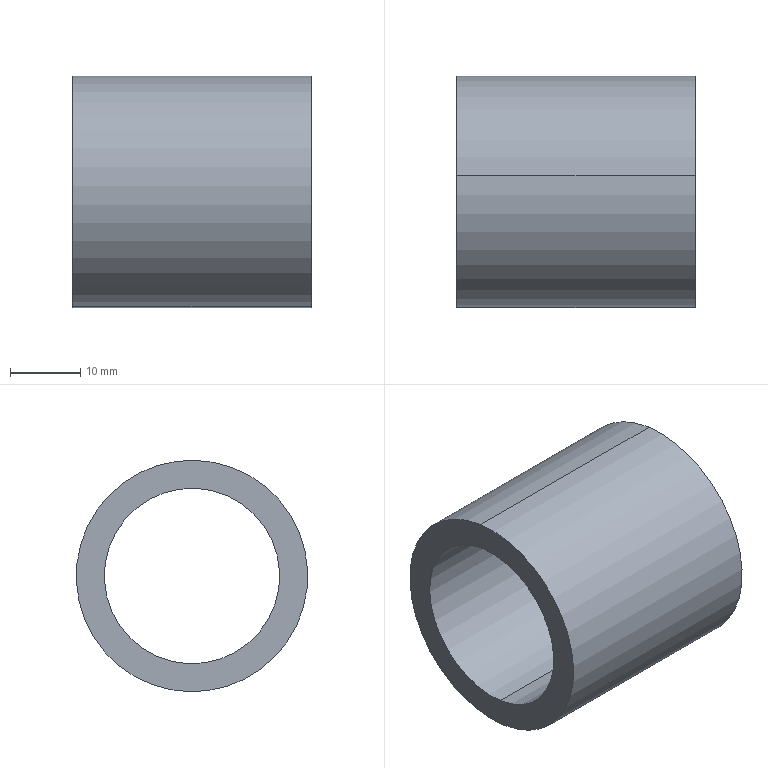Component | SolidWorks | 4-12-12ClampingAxisAssembly-1_4-12-7ClampingAxisBearingInnerPad-1 | 1 solid | 6 faces | box 34 x 33 x 33 mm | volume 12390 mm3 | cylinder 4 | plane 2 | commonest cylinder face diameters 25 x2 33 x2
build123d program:
from build123d import *

# Parameters (mm, degrees)
SKETCH1_R      = 16.5
SKETCH1_R_2    = 12.5
EXTRUDE1_DEPTH = 34


with BuildPart() as part:
    # Sketch1 → Extrude1 (new body)
    with BuildSketch(Plane(origin=(0, 0, 0), x_dir=(1, 0, 0), z_dir=(0, 1, 0))):
        with Locations(Location((0, 0, 0), (0, 0, 270))):
            Circle(SKETCH1_R)
        with Locations(Location((0, 0, 0), (0, 0, 270))):
            Circle(SKETCH1_R_2, mode=Mode.SUBTRACT)
    extrude(amount=EXTRUDE1_DEPTH)


solid = part.part

# Placed as in the assembly
solid = solid.moved(Location((-67.809, -4.181, 0), (0, 0, 90)))
STEP:
#1=COLOUR_RGB('',0.7922,0.8196,0.9333);
#2=FILL_AREA_STYLE_COLOUR('',#1);
#3=FILL_AREA_STYLE('',(#2));
#4=SURFACE_STYLE_FILL_AREA(#3);
#5=SURFACE_SIDE_STYLE('',(#4));
#6=SURFACE_STYLE_USAGE(.BOTH.,#5);
#7=PRESENTATION_STYLE_ASSIGNMENT((#6));
#8=CARTESIAN_POINT('',(-4.008,-0.2322,-0.4875));
#9=VERTEX_POINT('',#8);
#10=CARTESIAN_POINT('',(-4.008,-0.09704,0.4875));
#11=VERTEX_POINT('',#10);
#12=CARTESIAN_POINT('',(-4.008,-0.1646,0.));
#13=DIRECTION('',(-1.,-0.,-0.));
#14=DIRECTION('',(0.,0.1373,0.9905));
#15=AXIS2_PLACEMENT_3D('',#12,#13,#14);
#16=CIRCLE('',#15,0.4921);
#17=EDGE_CURVE('',#9,#11,#16,.T.);
#18=ORIENTED_EDGE('',*,*,#17,.T.);
#19=CARTESIAN_POINT('',(-2.67,-0.09704,0.4875));
#20=VERTEX_POINT('',#19);
#21=CARTESIAN_POINT('',(-4.008,-0.09704,0.4875));
#22=DIRECTION('',(1.,0.,0.));
#23=VECTOR('',#22,39.37);
#24=LINE('',#21,#23);
#25=EDGE_CURVE('',#11,#20,#24,.T.);
#26=ORIENTED_EDGE('',*,*,#25,.T.);
#27=CARTESIAN_POINT('',(-2.67,-0.2322,-0.4875));
#28=VERTEX_POINT('',#27);
#29=CARTESIAN_POINT('',(-2.67,-0.1646,0.));
#30=DIRECTION('',(-1.,-0.,-0.));
#31=DIRECTION('',(0.,0.1373,0.9905));
#32=AXIS2_PLACEMENT_3D('',#29,#30,#31);
#33=CIRCLE('',#32,0.4921);
#34=EDGE_CURVE('',#28,#20,#33,.T.);
#35=ORIENTED_EDGE('',*,*,#34,.F.);
#36=CARTESIAN_POINT('',(-4.008,-0.2322,-0.4875));
#37=DIRECTION('',(1.,0.,0.));
#38=VECTOR('',#37,39.37);
#39=LINE('',#36,#38);
#40=EDGE_CURVE('',#9,#28,#39,.T.);
#41=ORIENTED_EDGE('',*,*,#40,.F.);
#42=EDGE_LOOP('',(#18,#26,#35,#41));
#43=FACE_OUTER_BOUND('',#42,.T.);
#44=CARTESIAN_POINT('',(-4.008,-0.1646,0.));
#45=DIRECTION('',(1.,0.,0.));
#46=DIRECTION('',(0.,-0.1373,-0.9905));
#47=AXIS2_PLACEMENT_3D('',#44,#45,#46);
#48=CYLINDRICAL_SURFACE('',#47,0.4921);
#49=ADVANCED_FACE('',(#43),#48,.F.);
#50=CARTESIAN_POINT('',(-4.008,-0.07542,0.6435));
#51=VERTEX_POINT('',#50);
#52=CARTESIAN_POINT('',(-4.008,-0.2538,-0.6435));
#53=VERTEX_POINT('',#52);
#54=CARTESIAN_POINT('',(-4.008,-0.1646,0.));
#55=DIRECTION('',(-1.,-0.,-0.));
#56=DIRECTION('',(0.,0.1373,0.9905));
#57=AXIS2_PLACEMENT_3D('',#54,#55,#56);
#58=CIRCLE('',#57,0.6496);
#59=EDGE_CURVE('',#51,#53,#58,.T.);
#60=ORIENTED_EDGE('',*,*,#59,.F.);
#61=CARTESIAN_POINT('',(-2.67,-0.07542,0.6435));
#62=VERTEX_POINT('',#61);
#63=CARTESIAN_POINT('',(-4.008,-0.07542,0.6435));
#64=DIRECTION('',(1.,0.,0.));
#65=VECTOR('',#64,39.37);
#66=LINE('',#63,#65);
#67=EDGE_CURVE('',#51,#62,#66,.T.);
#68=ORIENTED_EDGE('',*,*,#67,.T.);
#69=CARTESIAN_POINT('',(-2.67,-0.2538,-0.6435));
#70=VERTEX_POINT('',#69);
#71=CARTESIAN_POINT('',(-2.67,-0.1646,0.));
#72=DIRECTION('',(-1.,-0.,-0.));
#73=DIRECTION('',(0.,0.1373,0.9905));
#74=AXIS2_PLACEMENT_3D('',#71,#72,#73);
#75=CIRCLE('',#74,0.6496);
#76=EDGE_CURVE('',#62,#70,#75,.T.);
#77=ORIENTED_EDGE('',*,*,#76,.T.);
#78=CARTESIAN_POINT('',(-4.008,-0.2538,-0.6435));
#79=DIRECTION('',(1.,0.,0.));
#80=VECTOR('',#79,39.37);
#81=LINE('',#78,#80);
#82=EDGE_CURVE('',#53,#70,#81,.T.);
#83=ORIENTED_EDGE('',*,*,#82,.F.);
#84=EDGE_LOOP('',(#60,#68,#77,#83));
#85=FACE_OUTER_BOUND('',#84,.T.);
#86=CARTESIAN_POINT('',(-4.008,-0.1646,0.));
#87=DIRECTION('',(1.,0.,0.));
#88=DIRECTION('',(0.,-0.1373,-0.9905));
#89=AXIS2_PLACEMENT_3D('',#86,#87,#88);
#90=CYLINDRICAL_SURFACE('',#89,0.6496);
#91=ADVANCED_FACE('',(#85),#90,.T.);
#92=CARTESIAN_POINT('',(-4.008,-0.1646,0.));
#93=DIRECTION('',(-1.,-0.,-0.));
#94=DIRECTION('',(0.,0.1373,0.9905));
#95=AXIS2_PLACEMENT_3D('',#92,#93,#94);
#96=CIRCLE('',#95,0.6496);
#97=EDGE_CURVE('',#53,#51,#96,.T.);
#98=ORIENTED_EDGE('',*,*,#97,.T.);
#99=ORIENTED_EDGE('',*,*,#59,.T.);
#100=EDGE_LOOP('',(#98,#99));
#101=FACE_OUTER_BOUND('',#100,.T.);
#102=ORIENTED_EDGE('',*,*,#17,.F.);
#103=CARTESIAN_POINT('',(-4.008,-0.1646,0.));
#104=DIRECTION('',(-1.,-0.,-0.));
#105=DIRECTION('',(0.,0.1373,0.9905));
#106=AXIS2_PLACEMENT_3D('',#103,#104,#105);
#107=CIRCLE('',#106,0.4921);
#108=EDGE_CURVE('',#11,#9,#107,.T.);
#109=ORIENTED_EDGE('',*,*,#108,.F.);
#110=EDGE_LOOP('',(#102,#109));
#111=FACE_BOUND('',#110,.T.);
#112=CARTESIAN_POINT('',(-4.008,-0.1646,0.));
#113=DIRECTION('',(-1.,-0.,-0.));
#114=DIRECTION('',(-0.,0.1373,0.9905));
#115=AXIS2_PLACEMENT_3D('',#112,#113,#114);
#116=PLANE('',#115);
#117=ADVANCED_FACE('',(#101,#111),#116,.T.);
#118=CARTESIAN_POINT('',(-2.67,-0.1646,0.));
#119=DIRECTION('',(-1.,-0.,-0.));
#120=DIRECTION('',(0.,0.1373,0.9905));
#121=AXIS2_PLACEMENT_3D('',#118,#119,#120);
#122=CIRCLE('',#121,0.6496);
#123=EDGE_CURVE('',#70,#62,#122,.T.);
#124=ORIENTED_EDGE('',*,*,#123,.F.);
#125=ORIENTED_EDGE('',*,*,#76,.F.);
#126=EDGE_LOOP('',(#124,#125));
#127=FACE_OUTER_BOUND('',#126,.T.);
#128=ORIENTED_EDGE('',*,*,#34,.T.);
#129=CARTESIAN_POINT('',(-2.67,-0.1646,0.));
#130=DIRECTION('',(-1.,-0.,-0.));
#131=DIRECTION('',(0.,0.1373,0.9905));
#132=AXIS2_PLACEMENT_3D('',#129,#130,#131);
#133=CIRCLE('',#132,0.4921);
#134=EDGE_CURVE('',#20,#28,#133,.T.);
#135=ORIENTED_EDGE('',*,*,#134,.T.);
#136=EDGE_LOOP('',(#128,#135));
#137=FACE_BOUND('',#136,.T.);
#138=CARTESIAN_POINT('',(-2.67,-0.1646,0.));
#139=DIRECTION('',(-1.,-0.,-0.));
#140=DIRECTION('',(-0.,0.1373,0.9905));
#141=AXIS2_PLACEMENT_3D('',#138,#139,#140);
#142=PLANE('',#141);
#143=ADVANCED_FACE('',(#127,#137),#142,.F.);
#144=ORIENTED_EDGE('',*,*,#67,.F.);
#145=ORIENTED_EDGE('',*,*,#97,.F.);
#146=ORIENTED_EDGE('',*,*,#82,.T.);
#147=ORIENTED_EDGE('',*,*,#123,.T.);
#148=EDGE_LOOP('',(#144,#145,#146,#147));
#149=FACE_OUTER_BOUND('',#148,.T.);
#150=CARTESIAN_POINT('',(-4.008,-0.1646,0.));
#151=DIRECTION('',(1.,0.,0.));
#152=DIRECTION('',(0.,-0.1373,-0.9905));
#153=AXIS2_PLACEMENT_3D('',#150,#151,#152);
#154=CYLINDRICAL_SURFACE('',#153,0.6496);
#155=ADVANCED_FACE('',(#149),#154,.T.);
#156=ORIENTED_EDGE('',*,*,#25,.F.);
#157=ORIENTED_EDGE('',*,*,#108,.T.);
#158=ORIENTED_EDGE('',*,*,#40,.T.);
#159=ORIENTED_EDGE('',*,*,#134,.F.);
#160=EDGE_LOOP('',(#156,#157,#158,#159));
#161=FACE_OUTER_BOUND('',#160,.T.);
#162=CARTESIAN_POINT('',(-4.008,-0.1646,0.));
#163=DIRECTION('',(1.,0.,0.));
#164=DIRECTION('',(0.,-0.1373,-0.9905));
#165=AXIS2_PLACEMENT_3D('',#162,#163,#164);
#166=CYLINDRICAL_SURFACE('',#165,0.4921);
#167=ADVANCED_FACE('',(#161),#166,.F.);
#168=CLOSED_SHELL('',(#49,#91,#117,#143,#155,#167));
#169=MANIFOLD_SOLID_BREP('',#168);
#170=STYLED_ITEM('',(#7),#169);
#171=(LENGTH_UNIT()NAMED_UNIT(*)SI_UNIT($,.METRE.));
#172=LENGTH_MEASURE_WITH_UNIT(LENGTH_MEASURE(0.0254),#171);
#173=DIMENSIONAL_EXPONENTS(1.,0.,0.,0.,0.,0.,0.);
#174=(CONVERSION_BASED_UNIT('',#172)LENGTH_UNIT()NAMED_UNIT(#173));
#175=UNCERTAINTY_MEASURE_WITH_UNIT(LENGTH_MEASURE(0.00001),#174,'','');
#176=(NAMED_UNIT(*)PLANE_ANGLE_UNIT()SI_UNIT($,.RADIAN.));
#177=(NAMED_UNIT(*)SI_UNIT($,.STERADIAN.)SOLID_ANGLE_UNIT());
#178=(GEOMETRIC_REPRESENTATION_CONTEXT(3)GLOBAL_UNCERTAINTY_ASSIGNED_CONTEXT((#175))GLOBAL_UNIT_ASSIGNED_CONTEXT((#174,#176,#177))REPRESENTATION_CONTEXT('',''));
#179=MECHANICAL_DESIGN_GEOMETRIC_PRESENTATION_REPRESENTATION('',(#170),#178);
#180=PRESENTATION_LAYER_ASSIGNMENT('','',(#170));
#181=CARTESIAN_POINT('',(0.,0.,0.));
#182=DIRECTION('',(0.,0.,1.));
#183=DIRECTION('',(1.,0.,0.));
#184=AXIS2_PLACEMENT_3D('',#181,#182,#183);
#185=(LENGTH_UNIT()NAMED_UNIT(*)SI_UNIT($,.METRE.));
#186=LENGTH_MEASURE_WITH_UNIT(LENGTH_MEASURE(0.0254),#185);
#187=DIMENSIONAL_EXPONENTS(1.,0.,0.,0.,0.,0.,0.);
#188=(CONVERSION_BASED_UNIT('',#186)LENGTH_UNIT()NAMED_UNIT(#187));
#189=UNCERTAINTY_MEASURE_WITH_UNIT(LENGTH_MEASURE(0.00001),#188,'','');
#190=(NAMED_UNIT(*)PLANE_ANGLE_UNIT()SI_UNIT($,.RADIAN.));
#191=(NAMED_UNIT(*)SI_UNIT($,.STERADIAN.)SOLID_ANGLE_UNIT());
#192=(GEOMETRIC_REPRESENTATION_CONTEXT(3)GLOBAL_UNCERTAINTY_ASSIGNED_CONTEXT((#189))GLOBAL_UNIT_ASSIGNED_CONTEXT((#188,#190,#191))REPRESENTATION_CONTEXT('',''));
#193=ADVANCED_BREP_SHAPE_REPRESENTATION('',(#169,#184),#192);